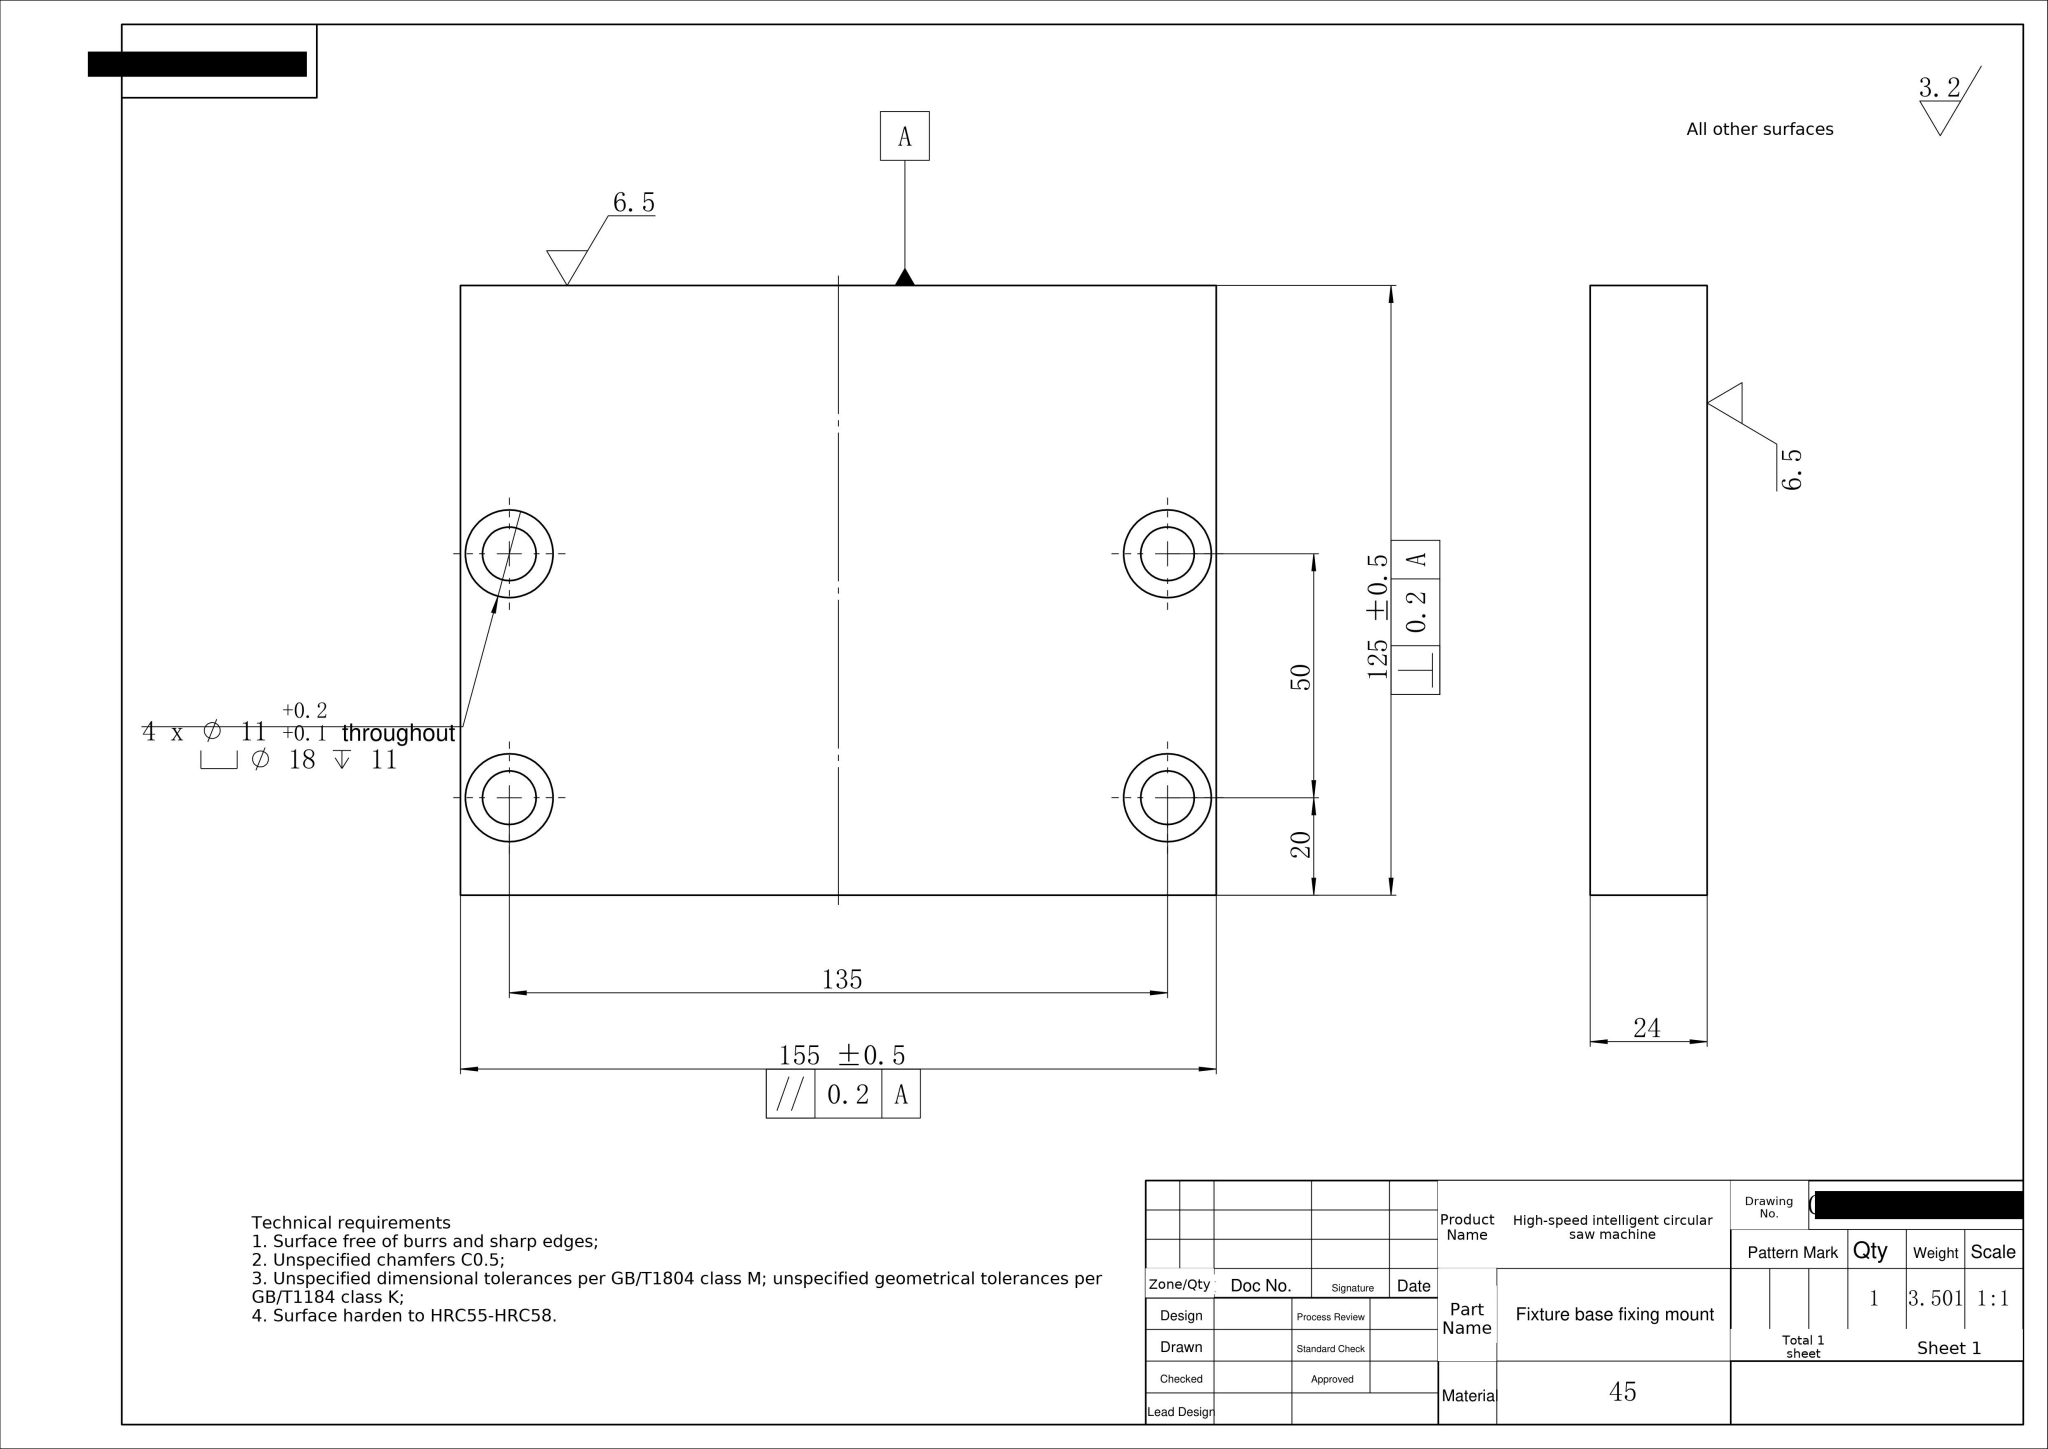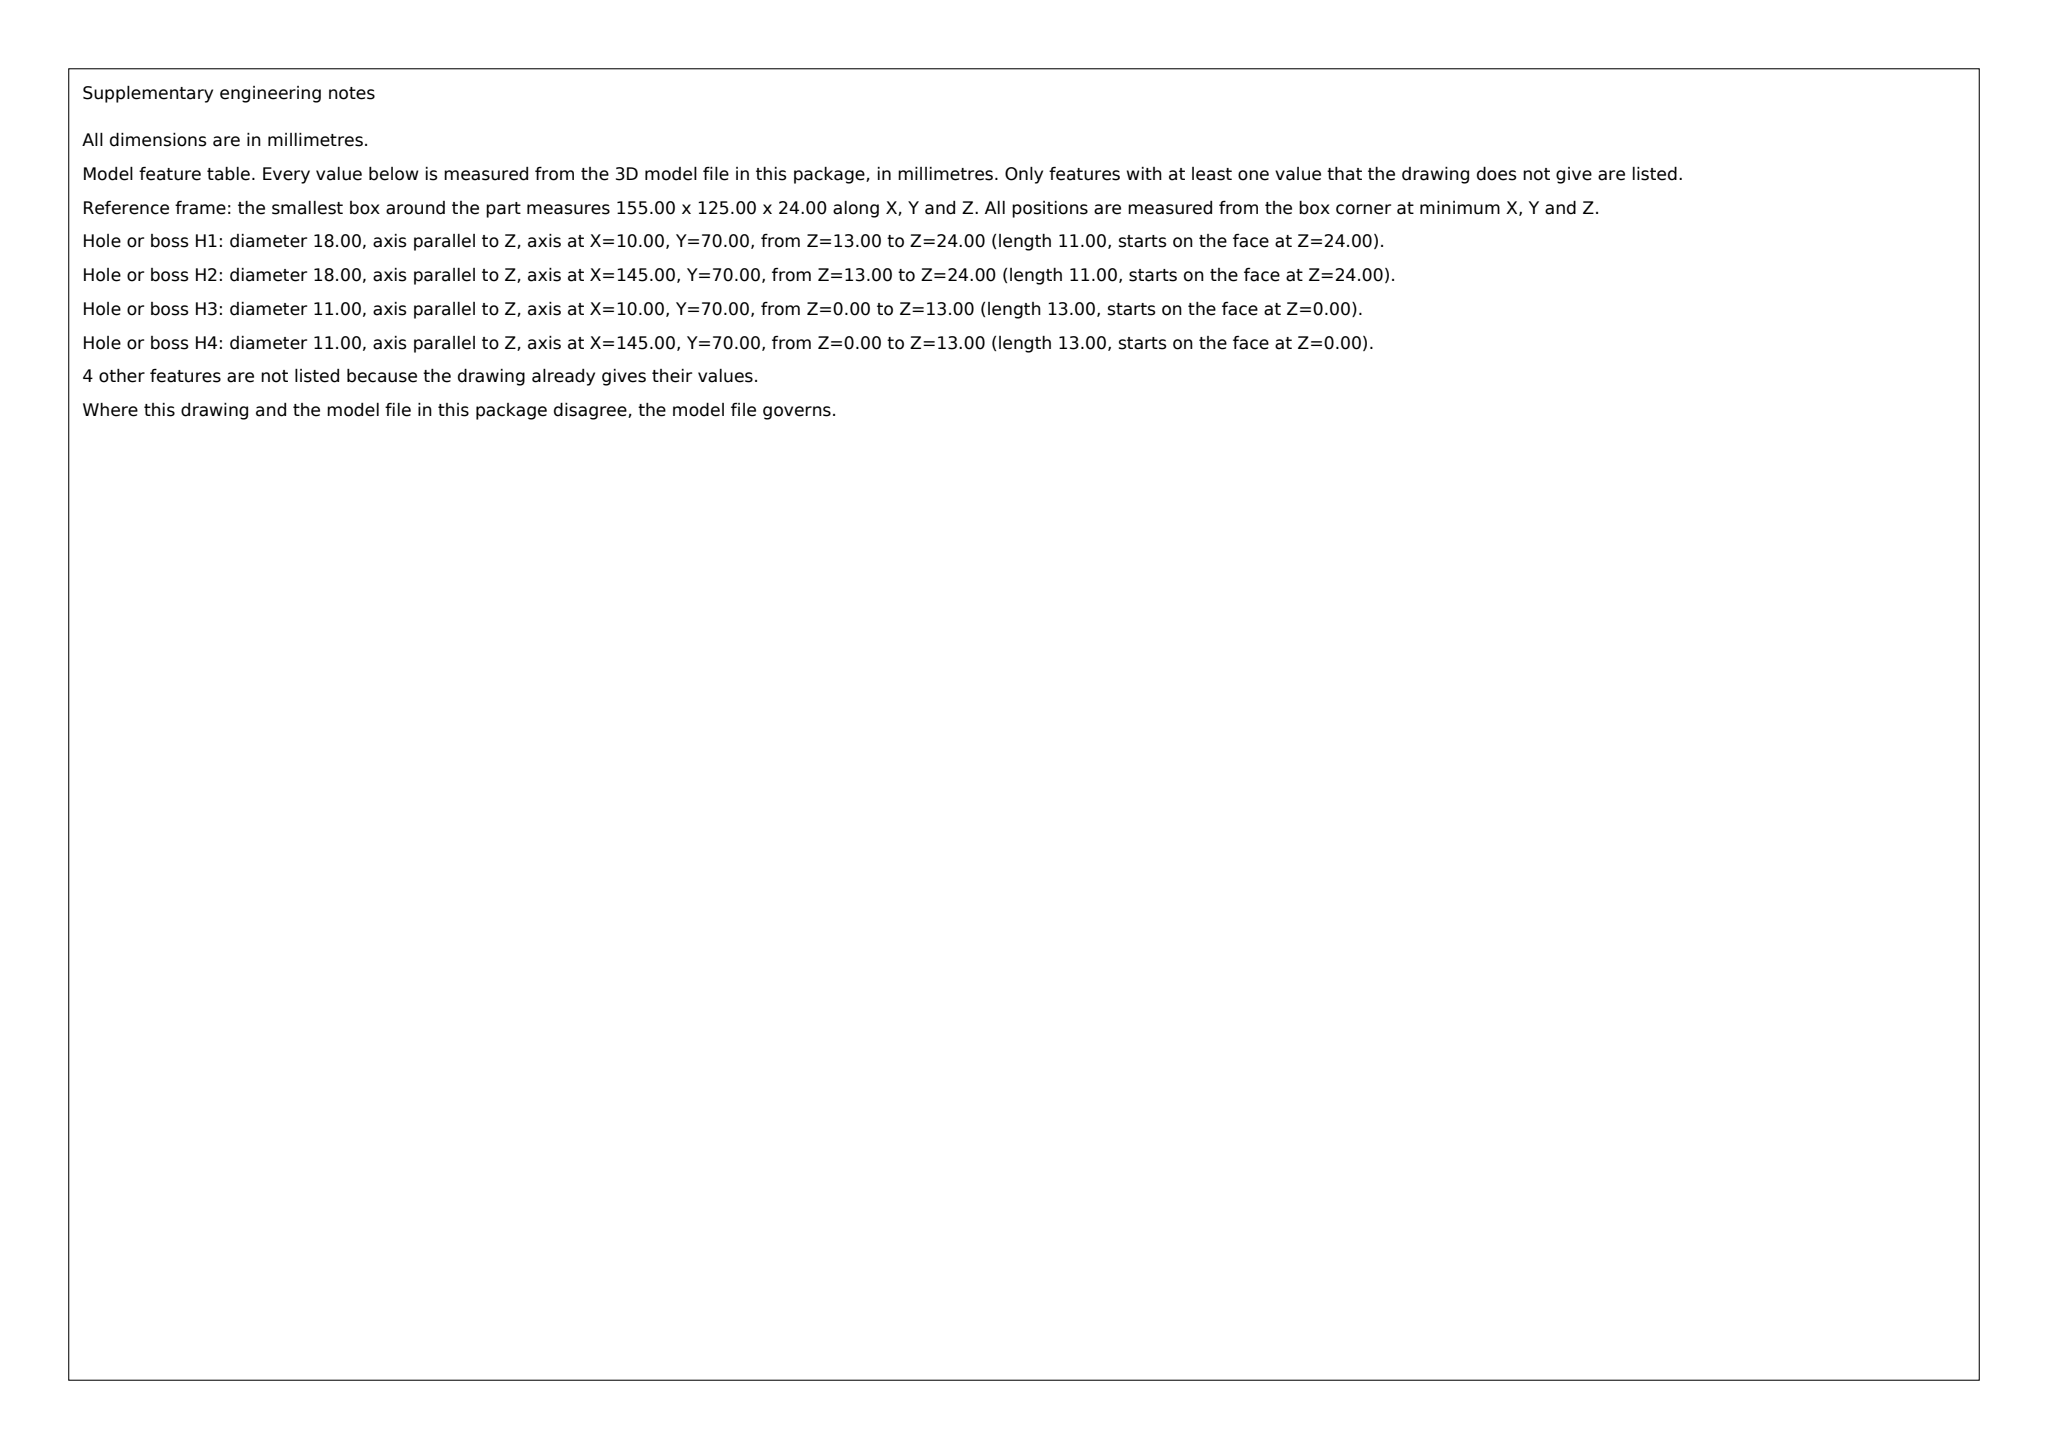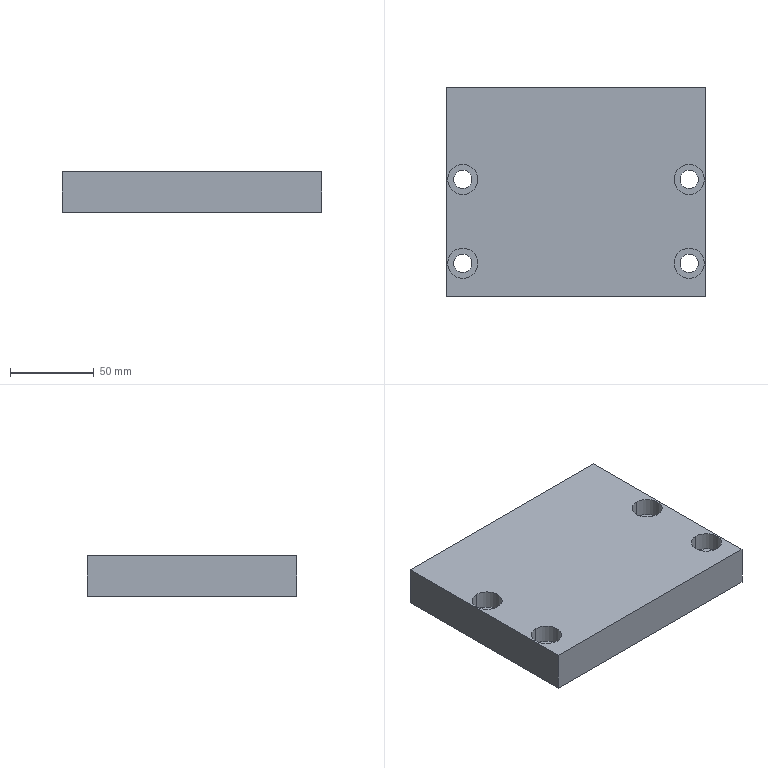Part | SolidWorks | mm | material 45 | 1 solid | 26 faces | box 155 x 125 x 24 mm | volume 448862 mm3 | cylinder 16 | plane 10 | commonest cylinder face diameters 18 x8 11 x8
build123d program:
from build123d import *

# Parameters (mm, degrees)
SKETCH1_W                                          = 24
SKETCH1_H                                          = 125
BOSS_EXTRUDE1_DEPTH                                = 155
HOLE_SIZE_ACCORDING_TO_TYPE_1_OF_HEXAG_D           = 11
HOLE_SIZE_ACCORDING_TO_TYPE_1_OF_HEXAG_CBORE_D     = 18
HOLE_SIZE_ACCORDING_TO_TYPE_1_OF_HEXAG_CBORE_DEPTH = 11


with BuildPart() as part:
    # Sketch1 → Boss-Extrude1 (new body)
    with BuildSketch(Plane(origin=(0, 0, 0), x_dir=(0, 0, -1), z_dir=(1, 0, 0))):
        with Locations((12, 62.5)):
            Rectangle(SKETCH1_W, SKETCH1_H)
    extrude(amount=BOSS_EXTRUDE1_DEPTH)

    # Hole Size _According to_ Type 1 of Hexag (through all)
    with Locations(Plane(origin=(10, 70, 0), x_dir=(1, 0, 0), z_dir=(0, 0, 1))):
        with Locations((0, 0), (0, -50), (135, 0), (135, -50)):
            CounterBoreHole(HOLE_SIZE_ACCORDING_TO_TYPE_1_OF_HEXAG_D / 2, HOLE_SIZE_ACCORDING_TO_TYPE_1_OF_HEXAG_CBORE_D / 2, HOLE_SIZE_ACCORDING_TO_TYPE_1_OF_HEXAG_CBORE_DEPTH)


solid = part.part
STEP:
#1=CARTESIAN_POINT('',(10.,79.,-11.));
#2=VERTEX_POINT('',#1);
#3=CARTESIAN_POINT('',(10.,61.,-11.));
#4=VERTEX_POINT('',#3);
#5=CARTESIAN_POINT('',(10.,70.,-11.));
#6=DIRECTION('',(0.,0.,1.));
#7=DIRECTION('',(0.,-1.,0.));
#8=AXIS2_PLACEMENT_3D('',#5,#6,#7);
#9=CIRCLE('',#8,9.);
#10=EDGE_CURVE('',#2,#4,#9,.T.);
#11=ORIENTED_EDGE('',*,*,#10,.F.);
#12=CARTESIAN_POINT('',(10.,79.,-0.));
#13=VERTEX_POINT('',#12);
#14=CARTESIAN_POINT('',(10.,79.,-0.));
#15=DIRECTION('',(0.,0.,1.));
#16=VECTOR('',#15,1000.);
#17=LINE('',#14,#16);
#18=EDGE_CURVE('',#2,#13,#17,.T.);
#19=ORIENTED_EDGE('',*,*,#18,.T.);
#20=CARTESIAN_POINT('',(10.,61.,0.));
#21=VERTEX_POINT('',#20);
#22=CARTESIAN_POINT('',(10.,70.,0.));
#23=DIRECTION('',(0.,0.,1.));
#24=DIRECTION('',(0.,-1.,0.));
#25=AXIS2_PLACEMENT_3D('',#22,#23,#24);
#26=CIRCLE('',#25,9.);
#27=EDGE_CURVE('',#13,#21,#26,.T.);
#28=ORIENTED_EDGE('',*,*,#27,.T.);
#29=CARTESIAN_POINT('',(10.,61.,0.));
#30=DIRECTION('',(0.,0.,1.));
#31=VECTOR('',#30,1000.);
#32=LINE('',#29,#31);
#33=EDGE_CURVE('',#4,#21,#32,.T.);
#34=ORIENTED_EDGE('',*,*,#33,.F.);
#35=EDGE_LOOP('',(#11,#19,#28,#34));
#36=FACE_OUTER_BOUND('',#35,.T.);
#37=CARTESIAN_POINT('',(10.,70.,0.));
#38=DIRECTION('',(0.,0.,1.));
#39=DIRECTION('',(0.,-1.,0.));
#40=AXIS2_PLACEMENT_3D('',#37,#38,#39);
#41=CYLINDRICAL_SURFACE('',#40,9.);
#42=ADVANCED_FACE('',(#36),#41,.F.);
#43=CARTESIAN_POINT('',(10.,75.5,-24.));
#44=VERTEX_POINT('',#43);
#45=CARTESIAN_POINT('',(10.,64.5,-24.));
#46=VERTEX_POINT('',#45);
#47=CARTESIAN_POINT('',(10.,70.,-24.));
#48=DIRECTION('',(0.,0.,1.));
#49=DIRECTION('',(0.,-1.,0.));
#50=AXIS2_PLACEMENT_3D('',#47,#48,#49);
#51=CIRCLE('',#50,5.5);
#52=EDGE_CURVE('',#44,#46,#51,.T.);
#53=ORIENTED_EDGE('',*,*,#52,.F.);
#54=CARTESIAN_POINT('',(10.,75.5,-11.));
#55=VERTEX_POINT('',#54);
#56=CARTESIAN_POINT('',(10.,75.5,-0.));
#57=DIRECTION('',(0.,0.,1.));
#58=VECTOR('',#57,1000.);
#59=LINE('',#56,#58);
#60=EDGE_CURVE('',#44,#55,#59,.T.);
#61=ORIENTED_EDGE('',*,*,#60,.T.);
#62=CARTESIAN_POINT('',(10.,64.5,-11.));
#63=VERTEX_POINT('',#62);
#64=CARTESIAN_POINT('',(10.,70.,-11.));
#65=DIRECTION('',(0.,0.,1.));
#66=DIRECTION('',(0.,-1.,0.));
#67=AXIS2_PLACEMENT_3D('',#64,#65,#66);
#68=CIRCLE('',#67,5.5);
#69=EDGE_CURVE('',#55,#63,#68,.T.);
#70=ORIENTED_EDGE('',*,*,#69,.T.);
#71=CARTESIAN_POINT('',(10.,64.5,0.));
#72=DIRECTION('',(0.,0.,1.));
#73=VECTOR('',#72,1000.);
#74=LINE('',#71,#73);
#75=EDGE_CURVE('',#46,#63,#74,.T.);
#76=ORIENTED_EDGE('',*,*,#75,.F.);
#77=EDGE_LOOP('',(#53,#61,#70,#76));
#78=FACE_OUTER_BOUND('',#77,.T.);
#79=CARTESIAN_POINT('',(10.,70.,0.));
#80=DIRECTION('',(0.,0.,1.));
#81=DIRECTION('',(0.,-1.,0.));
#82=AXIS2_PLACEMENT_3D('',#79,#80,#81);
#83=CYLINDRICAL_SURFACE('',#82,5.5);
#84=ADVANCED_FACE('',(#78),#83,.F.);
#85=CARTESIAN_POINT('',(10.,29.,-11.));
#86=VERTEX_POINT('',#85);
#87=CARTESIAN_POINT('',(10.,11.,-11.));
#88=VERTEX_POINT('',#87);
#89=CARTESIAN_POINT('',(10.,20.,-11.));
#90=DIRECTION('',(0.,0.,1.));
#91=DIRECTION('',(0.,-1.,0.));
#92=AXIS2_PLACEMENT_3D('',#89,#90,#91);
#93=CIRCLE('',#92,9.);
#94=EDGE_CURVE('',#86,#88,#93,.T.);
#95=ORIENTED_EDGE('',*,*,#94,.F.);
#96=CARTESIAN_POINT('',(10.,29.,-0.));
#97=VERTEX_POINT('',#96);
#98=CARTESIAN_POINT('',(10.,29.,-0.));
#99=DIRECTION('',(0.,0.,1.));
#100=VECTOR('',#99,1000.);
#101=LINE('',#98,#100);
#102=EDGE_CURVE('',#86,#97,#101,.T.);
#103=ORIENTED_EDGE('',*,*,#102,.T.);
#104=CARTESIAN_POINT('',(10.,11.,0.));
#105=VERTEX_POINT('',#104);
#106=CARTESIAN_POINT('',(10.,20.,0.));
#107=DIRECTION('',(0.,0.,1.));
#108=DIRECTION('',(0.,-1.,0.));
#109=AXIS2_PLACEMENT_3D('',#106,#107,#108);
#110=CIRCLE('',#109,9.);
#111=EDGE_CURVE('',#97,#105,#110,.T.);
#112=ORIENTED_EDGE('',*,*,#111,.T.);
#113=CARTESIAN_POINT('',(10.,11.,0.));
#114=DIRECTION('',(0.,0.,1.));
#115=VECTOR('',#114,1000.);
#116=LINE('',#113,#115);
#117=EDGE_CURVE('',#88,#105,#116,.T.);
#118=ORIENTED_EDGE('',*,*,#117,.F.);
#119=EDGE_LOOP('',(#95,#103,#112,#118));
#120=FACE_OUTER_BOUND('',#119,.T.);
#121=CARTESIAN_POINT('',(10.,20.,0.));
#122=DIRECTION('',(0.,0.,1.));
#123=DIRECTION('',(0.,-1.,0.));
#124=AXIS2_PLACEMENT_3D('',#121,#122,#123);
#125=CYLINDRICAL_SURFACE('',#124,9.);
#126=ADVANCED_FACE('',(#120),#125,.F.);
#127=CARTESIAN_POINT('',(10.,25.5,-24.));
#128=VERTEX_POINT('',#127);
#129=CARTESIAN_POINT('',(10.,14.5,-24.));
#130=VERTEX_POINT('',#129);
#131=CARTESIAN_POINT('',(10.,20.,-24.));
#132=DIRECTION('',(0.,0.,1.));
#133=DIRECTION('',(0.,-1.,0.));
#134=AXIS2_PLACEMENT_3D('',#131,#132,#133);
#135=CIRCLE('',#134,5.5);
#136=EDGE_CURVE('',#128,#130,#135,.T.);
#137=ORIENTED_EDGE('',*,*,#136,.F.);
#138=CARTESIAN_POINT('',(10.,25.5,-11.));
#139=VERTEX_POINT('',#138);
#140=CARTESIAN_POINT('',(10.,25.5,-0.));
#141=DIRECTION('',(0.,0.,1.));
#142=VECTOR('',#141,1000.);
#143=LINE('',#140,#142);
#144=EDGE_CURVE('',#128,#139,#143,.T.);
#145=ORIENTED_EDGE('',*,*,#144,.T.);
#146=CARTESIAN_POINT('',(10.,14.5,-11.));
#147=VERTEX_POINT('',#146);
#148=CARTESIAN_POINT('',(10.,20.,-11.));
#149=DIRECTION('',(0.,0.,1.));
#150=DIRECTION('',(0.,-1.,0.));
#151=AXIS2_PLACEMENT_3D('',#148,#149,#150);
#152=CIRCLE('',#151,5.5);
#153=EDGE_CURVE('',#139,#147,#152,.T.);
#154=ORIENTED_EDGE('',*,*,#153,.T.);
#155=CARTESIAN_POINT('',(10.,14.5,0.));
#156=DIRECTION('',(0.,0.,1.));
#157=VECTOR('',#156,1000.);
#158=LINE('',#155,#157);
#159=EDGE_CURVE('',#130,#147,#158,.T.);
#160=ORIENTED_EDGE('',*,*,#159,.F.);
#161=EDGE_LOOP('',(#137,#145,#154,#160));
#162=FACE_OUTER_BOUND('',#161,.T.);
#163=CARTESIAN_POINT('',(10.,20.,0.));
#164=DIRECTION('',(0.,0.,1.));
#165=DIRECTION('',(0.,-1.,0.));
#166=AXIS2_PLACEMENT_3D('',#163,#164,#165);
#167=CYLINDRICAL_SURFACE('',#166,5.5);
#168=ADVANCED_FACE('',(#162),#167,.F.);
#169=CARTESIAN_POINT('',(145.,79.,-11.));
#170=VERTEX_POINT('',#169);
#171=CARTESIAN_POINT('',(145.,61.,-11.));
#172=VERTEX_POINT('',#171);
#173=CARTESIAN_POINT('',(145.,70.,-11.));
#174=DIRECTION('',(0.,0.,1.));
#175=DIRECTION('',(0.,-1.,0.));
#176=AXIS2_PLACEMENT_3D('',#173,#174,#175);
#177=CIRCLE('',#176,9.);
#178=EDGE_CURVE('',#170,#172,#177,.T.);
#179=ORIENTED_EDGE('',*,*,#178,.F.);
#180=CARTESIAN_POINT('',(145.,79.,-0.));
#181=VERTEX_POINT('',#180);
#182=CARTESIAN_POINT('',(145.,79.,-0.));
#183=DIRECTION('',(0.,0.,1.));
#184=VECTOR('',#183,1000.);
#185=LINE('',#182,#184);
#186=EDGE_CURVE('',#170,#181,#185,.T.);
#187=ORIENTED_EDGE('',*,*,#186,.T.);
#188=CARTESIAN_POINT('',(145.,61.,0.));
#189=VERTEX_POINT('',#188);
#190=CARTESIAN_POINT('',(145.,70.,0.));
#191=DIRECTION('',(0.,0.,1.));
#192=DIRECTION('',(0.,-1.,0.));
#193=AXIS2_PLACEMENT_3D('',#190,#191,#192);
#194=CIRCLE('',#193,9.);
#195=EDGE_CURVE('',#181,#189,#194,.T.);
#196=ORIENTED_EDGE('',*,*,#195,.T.);
#197=CARTESIAN_POINT('',(145.,61.,0.));
#198=DIRECTION('',(0.,0.,1.));
#199=VECTOR('',#198,1000.);
#200=LINE('',#197,#199);
#201=EDGE_CURVE('',#172,#189,#200,.T.);
#202=ORIENTED_EDGE('',*,*,#201,.F.);
#203=EDGE_LOOP('',(#179,#187,#196,#202));
#204=FACE_OUTER_BOUND('',#203,.T.);
#205=CARTESIAN_POINT('',(145.,70.,0.));
#206=DIRECTION('',(0.,0.,1.));
#207=DIRECTION('',(0.,-1.,0.));
#208=AXIS2_PLACEMENT_3D('',#205,#206,#207);
#209=CYLINDRICAL_SURFACE('',#208,9.);
#210=ADVANCED_FACE('',(#204),#209,.F.);
#211=CARTESIAN_POINT('',(145.,75.5,-24.));
#212=VERTEX_POINT('',#211);
#213=CARTESIAN_POINT('',(145.,64.5,-24.));
#214=VERTEX_POINT('',#213);
#215=CARTESIAN_POINT('',(145.,70.,-24.));
#216=DIRECTION('',(0.,0.,1.));
#217=DIRECTION('',(0.,-1.,0.));
#218=AXIS2_PLACEMENT_3D('',#215,#216,#217);
#219=CIRCLE('',#218,5.5);
#220=EDGE_CURVE('',#212,#214,#219,.T.);
#221=ORIENTED_EDGE('',*,*,#220,.F.);
#222=CARTESIAN_POINT('',(145.,75.5,-11.));
#223=VERTEX_POINT('',#222);
#224=CARTESIAN_POINT('',(145.,75.5,-0.));
#225=DIRECTION('',(0.,0.,1.));
#226=VECTOR('',#225,1000.);
#227=LINE('',#224,#226);
#228=EDGE_CURVE('',#212,#223,#227,.T.);
#229=ORIENTED_EDGE('',*,*,#228,.T.);
#230=CARTESIAN_POINT('',(145.,64.5,-11.));
#231=VERTEX_POINT('',#230);
#232=CARTESIAN_POINT('',(145.,70.,-11.));
#233=DIRECTION('',(0.,0.,1.));
#234=DIRECTION('',(0.,-1.,0.));
#235=AXIS2_PLACEMENT_3D('',#232,#233,#234);
#236=CIRCLE('',#235,5.5);
#237=EDGE_CURVE('',#223,#231,#236,.T.);
#238=ORIENTED_EDGE('',*,*,#237,.T.);
#239=CARTESIAN_POINT('',(145.,64.5,0.));
#240=DIRECTION('',(0.,0.,1.));
#241=VECTOR('',#240,1000.);
#242=LINE('',#239,#241);
#243=EDGE_CURVE('',#214,#231,#242,.T.);
#244=ORIENTED_EDGE('',*,*,#243,.F.);
#245=EDGE_LOOP('',(#221,#229,#238,#244));
#246=FACE_OUTER_BOUND('',#245,.T.);
#247=CARTESIAN_POINT('',(145.,70.,0.));
#248=DIRECTION('',(0.,0.,1.));
#249=DIRECTION('',(0.,-1.,0.));
#250=AXIS2_PLACEMENT_3D('',#247,#248,#249);
#251=CYLINDRICAL_SURFACE('',#250,5.5);
#252=ADVANCED_FACE('',(#246),#251,.F.);
#253=CARTESIAN_POINT('',(145.,29.,-11.));
#254=VERTEX_POINT('',#253);
#255=CARTESIAN_POINT('',(145.,11.,-11.));
#256=VERTEX_POINT('',#255);
#257=CARTESIAN_POINT('',(145.,20.,-11.));
#258=DIRECTION('',(0.,0.,1.));
#259=DIRECTION('',(0.,-1.,0.));
#260=AXIS2_PLACEMENT_3D('',#257,#258,#259);
#261=CIRCLE('',#260,9.);
#262=EDGE_CURVE('',#254,#256,#261,.T.);
#263=ORIENTED_EDGE('',*,*,#262,.F.);
#264=CARTESIAN_POINT('',(145.,29.,-0.));
#265=VERTEX_POINT('',#264);
#266=CARTESIAN_POINT('',(145.,29.,-0.));
#267=DIRECTION('',(0.,0.,1.));
#268=VECTOR('',#267,1000.);
#269=LINE('',#266,#268);
#270=EDGE_CURVE('',#254,#265,#269,.T.);
#271=ORIENTED_EDGE('',*,*,#270,.T.);
#272=CARTESIAN_POINT('',(145.,11.,0.));
#273=VERTEX_POINT('',#272);
#274=CARTESIAN_POINT('',(145.,20.,0.));
#275=DIRECTION('',(0.,0.,1.));
#276=DIRECTION('',(0.,-1.,0.));
#277=AXIS2_PLACEMENT_3D('',#274,#275,#276);
#278=CIRCLE('',#277,9.);
#279=EDGE_CURVE('',#265,#273,#278,.T.);
#280=ORIENTED_EDGE('',*,*,#279,.T.);
#281=CARTESIAN_POINT('',(145.,11.,0.));
#282=DIRECTION('',(0.,0.,1.));
#283=VECTOR('',#282,1000.);
#284=LINE('',#281,#283);
#285=EDGE_CURVE('',#256,#273,#284,.T.);
#286=ORIENTED_EDGE('',*,*,#285,.F.);
#287=EDGE_LOOP('',(#263,#271,#280,#286));
#288=FACE_OUTER_BOUND('',#287,.T.);
#289=CARTESIAN_POINT('',(145.,20.,0.));
#290=DIRECTION('',(0.,0.,1.));
#291=DIRECTION('',(0.,-1.,0.));
#292=AXIS2_PLACEMENT_3D('',#289,#290,#291);
#293=CYLINDRICAL_SURFACE('',#292,9.);
#294=ADVANCED_FACE('',(#288),#293,.F.);
#295=CARTESIAN_POINT('',(145.,25.5,-24.));
#296=VERTEX_POINT('',#295);
#297=CARTESIAN_POINT('',(145.,14.5,-24.));
#298=VERTEX_POINT('',#297);
#299=CARTESIAN_POINT('',(145.,20.,-24.));
#300=DIRECTION('',(0.,0.,1.));
#301=DIRECTION('',(0.,-1.,0.));
#302=AXIS2_PLACEMENT_3D('',#299,#300,#301);
#303=CIRCLE('',#302,5.5);
#304=EDGE_CURVE('',#296,#298,#303,.T.);
#305=ORIENTED_EDGE('',*,*,#304,.F.);
#306=CARTESIAN_POINT('',(145.,25.5,-11.));
#307=VERTEX_POINT('',#306);
#308=CARTESIAN_POINT('',(145.,25.5,-0.));
#309=DIRECTION('',(0.,0.,1.));
#310=VECTOR('',#309,1000.);
#311=LINE('',#308,#310);
#312=EDGE_CURVE('',#296,#307,#311,.T.);
#313=ORIENTED_EDGE('',*,*,#312,.T.);
#314=CARTESIAN_POINT('',(145.,14.5,-11.));
#315=VERTEX_POINT('',#314);
#316=CARTESIAN_POINT('',(145.,20.,-11.));
#317=DIRECTION('',(0.,0.,1.));
#318=DIRECTION('',(0.,-1.,0.));
#319=AXIS2_PLACEMENT_3D('',#316,#317,#318);
#320=CIRCLE('',#319,5.5);
#321=EDGE_CURVE('',#307,#315,#320,.T.);
#322=ORIENTED_EDGE('',*,*,#321,.T.);
#323=CARTESIAN_POINT('',(145.,14.5,0.));
#324=DIRECTION('',(0.,0.,1.));
#325=VECTOR('',#324,1000.);
#326=LINE('',#323,#325);
#327=EDGE_CURVE('',#298,#315,#326,.T.);
#328=ORIENTED_EDGE('',*,*,#327,.F.);
#329=EDGE_LOOP('',(#305,#313,#322,#328));
#330=FACE_OUTER_BOUND('',#329,.T.);
#331=CARTESIAN_POINT('',(145.,20.,0.));
#332=DIRECTION('',(0.,0.,1.));
#333=DIRECTION('',(0.,-1.,0.));
#334=AXIS2_PLACEMENT_3D('',#331,#332,#333);
#335=CYLINDRICAL_SURFACE('',#334,5.5);
#336=ADVANCED_FACE('',(#330),#335,.F.);
#337=CARTESIAN_POINT('',(10.,70.,0.));
#338=DIRECTION('',(0.,0.,1.));
#339=DIRECTION('',(0.,-1.,0.));
#340=AXIS2_PLACEMENT_3D('',#337,#338,#339);
#341=CIRCLE('',#340,9.);
#342=EDGE_CURVE('',#21,#13,#341,.T.);
#343=ORIENTED_EDGE('',*,*,#342,.F.);
#344=ORIENTED_EDGE('',*,*,#27,.F.);
#345=EDGE_LOOP('',(#343,#344));
#346=FACE_BOUND('',#345,.T.);
#347=CARTESIAN_POINT('',(10.,20.,0.));
#348=DIRECTION('',(0.,0.,1.));
#349=DIRECTION('',(0.,-1.,0.));
#350=AXIS2_PLACEMENT_3D('',#347,#348,#349);
#351=CIRCLE('',#350,9.);
#352=EDGE_CURVE('',#105,#97,#351,.T.);
#353=ORIENTED_EDGE('',*,*,#352,.F.);
#354=ORIENTED_EDGE('',*,*,#111,.F.);
#355=EDGE_LOOP('',(#353,#354));
#356=FACE_BOUND('',#355,.T.);
#357=CARTESIAN_POINT('',(145.,70.,0.));
#358=DIRECTION('',(0.,0.,1.));
#359=DIRECTION('',(0.,-1.,0.));
#360=AXIS2_PLACEMENT_3D('',#357,#358,#359);
#361=CIRCLE('',#360,9.);
#362=EDGE_CURVE('',#189,#181,#361,.T.);
#363=ORIENTED_EDGE('',*,*,#362,.F.);
#364=ORIENTED_EDGE('',*,*,#195,.F.);
#365=EDGE_LOOP('',(#363,#364));
#366=FACE_BOUND('',#365,.T.);
#367=CARTESIAN_POINT('',(145.,20.,0.));
#368=DIRECTION('',(0.,0.,1.));
#369=DIRECTION('',(0.,-1.,0.));
#370=AXIS2_PLACEMENT_3D('',#367,#368,#369);
#371=CIRCLE('',#370,9.);
#372=EDGE_CURVE('',#273,#265,#371,.T.);
#373=ORIENTED_EDGE('',*,*,#372,.F.);
#374=ORIENTED_EDGE('',*,*,#279,.F.);
#375=EDGE_LOOP('',(#373,#374));
#376=FACE_BOUND('',#375,.T.);
#377=CARTESIAN_POINT('',(0.,125.,-0.));
#378=VERTEX_POINT('',#377);
#379=CARTESIAN_POINT('',(0.,0.,0.));
#380=VERTEX_POINT('',#379);
#381=CARTESIAN_POINT('',(0.,125.,-0.));
#382=DIRECTION('',(0.,-1.,0.));
#383=VECTOR('',#382,1000.);
#384=LINE('',#381,#383);
#385=EDGE_CURVE('',#378,#380,#384,.T.);
#386=ORIENTED_EDGE('',*,*,#385,.T.);
#387=CARTESIAN_POINT('',(155.,0.,0.));
#388=VERTEX_POINT('',#387);
#389=CARTESIAN_POINT('',(155.,0.,0.));
#390=DIRECTION('',(-1.,0.,0.));
#391=VECTOR('',#390,1000.);
#392=LINE('',#389,#391);
#393=EDGE_CURVE('',#388,#380,#392,.T.);
#394=ORIENTED_EDGE('',*,*,#393,.F.);
#395=CARTESIAN_POINT('',(155.,125.,-0.));
#396=VERTEX_POINT('',#395);
#397=CARTESIAN_POINT('',(155.,125.,-0.));
#398=DIRECTION('',(0.,-1.,0.));
#399=VECTOR('',#398,1000.);
#400=LINE('',#397,#399);
#401=EDGE_CURVE('',#396,#388,#400,.T.);
#402=ORIENTED_EDGE('',*,*,#401,.F.);
#403=CARTESIAN_POINT('',(155.,125.,-0.));
#404=DIRECTION('',(-1.,0.,0.));
#405=VECTOR('',#404,1000.);
#406=LINE('',#403,#405);
#407=EDGE_CURVE('',#396,#378,#406,.T.);
#408=ORIENTED_EDGE('',*,*,#407,.T.);
#409=EDGE_LOOP('',(#386,#394,#402,#408));
#410=FACE_OUTER_BOUND('',#409,.T.);
#411=CARTESIAN_POINT('',(155.,125.,-0.));
#412=DIRECTION('',(0.,-0.,-1.));
#413=DIRECTION('',(0.,1.,-0.));
#414=AXIS2_PLACEMENT_3D('',#411,#412,#413);
#415=PLANE('',#414);
#416=ADVANCED_FACE('',(#346,#356,#366,#376,#410),#415,.F.);
#417=CARTESIAN_POINT('',(0.,0.,-24.));
#418=VERTEX_POINT('',#417);
#419=CARTESIAN_POINT('',(0.,0.,0.));
#420=DIRECTION('',(0.,0.,-1.));
#421=VECTOR('',#420,1000.);
#422=LINE('',#419,#421);
#423=EDGE_CURVE('',#380,#418,#422,.T.);
#424=ORIENTED_EDGE('',*,*,#423,.T.);
#425=CARTESIAN_POINT('',(155.,0.,-24.));
#426=VERTEX_POINT('',#425);
#427=CARTESIAN_POINT('',(155.,0.,-24.));
#428=DIRECTION('',(-1.,0.,0.));
#429=VECTOR('',#428,1000.);
#430=LINE('',#427,#429);
#431=EDGE_CURVE('',#426,#418,#430,.T.);
#432=ORIENTED_EDGE('',*,*,#431,.F.);
#433=CARTESIAN_POINT('',(155.,0.,0.));
#434=DIRECTION('',(0.,0.,-1.));
#435=VECTOR('',#434,1000.);
#436=LINE('',#433,#435);
#437=EDGE_CURVE('',#388,#426,#436,.T.);
#438=ORIENTED_EDGE('',*,*,#437,.F.);
#439=ORIENTED_EDGE('',*,*,#393,.T.);
#440=EDGE_LOOP('',(#424,#432,#438,#439));
#441=FACE_OUTER_BOUND('',#440,.T.);
#442=CARTESIAN_POINT('',(155.,0.,0.));
#443=DIRECTION('',(0.,1.,0.));
#444=DIRECTION('',(0.,0.,1.));
#445=AXIS2_PLACEMENT_3D('',#442,#443,#444);
#446=PLANE('',#445);
#447=ADVANCED_FACE('',(#441),#446,.F.);
#448=CARTESIAN_POINT('',(10.,70.,-24.));
#449=DIRECTION('',(0.,0.,1.));
#450=DIRECTION('',(0.,-1.,0.));
#451=AXIS2_PLACEMENT_3D('',#448,#449,#450);
#452=CIRCLE('',#451,5.5);
#453=EDGE_CURVE('',#46,#44,#452,.T.);
#454=ORIENTED_EDGE('',*,*,#453,.T.);
#455=ORIENTED_EDGE('',*,*,#52,.T.);
#456=EDGE_LOOP('',(#454,#455));
#457=FACE_BOUND('',#456,.T.);
#458=CARTESIAN_POINT('',(10.,20.,-24.));
#459=DIRECTION('',(0.,0.,1.));
#460=DIRECTION('',(0.,-1.,0.));
#461=AXIS2_PLACEMENT_3D('',#458,#459,#460);
#462=CIRCLE('',#461,5.5);
#463=EDGE_CURVE('',#130,#128,#462,.T.);
#464=ORIENTED_EDGE('',*,*,#463,.T.);
#465=ORIENTED_EDGE('',*,*,#136,.T.);
#466=EDGE_LOOP('',(#464,#465));
#467=FACE_BOUND('',#466,.T.);
#468=CARTESIAN_POINT('',(145.,70.,-24.));
#469=DIRECTION('',(0.,0.,1.));
#470=DIRECTION('',(0.,-1.,0.));
#471=AXIS2_PLACEMENT_3D('',#468,#469,#470);
#472=CIRCLE('',#471,5.5);
#473=EDGE_CURVE('',#214,#212,#472,.T.);
#474=ORIENTED_EDGE('',*,*,#473,.T.);
#475=ORIENTED_EDGE('',*,*,#220,.T.);
#476=EDGE_LOOP('',(#474,#475));
#477=FACE_BOUND('',#476,.T.);
#478=CARTESIAN_POINT('',(145.,20.,-24.));
#479=DIRECTION('',(0.,0.,1.));
#480=DIRECTION('',(0.,-1.,0.));
#481=AXIS2_PLACEMENT_3D('',#478,#479,#480);
#482=CIRCLE('',#481,5.5);
#483=EDGE_CURVE('',#298,#296,#482,.T.);
#484=ORIENTED_EDGE('',*,*,#483,.T.);
#485=ORIENTED_EDGE('',*,*,#304,.T.);
#486=EDGE_LOOP('',(#484,#485));
#487=FACE_BOUND('',#486,.T.);
#488=CARTESIAN_POINT('',(0.,125.,-24.));
#489=VERTEX_POINT('',#488);
#490=CARTESIAN_POINT('',(0.,0.,-24.));
#491=DIRECTION('',(0.,1.,0.));
#492=VECTOR('',#491,1000.);
#493=LINE('',#490,#492);
#494=EDGE_CURVE('',#418,#489,#493,.T.);
#495=ORIENTED_EDGE('',*,*,#494,.T.);
#496=CARTESIAN_POINT('',(155.,125.,-24.));
#497=VERTEX_POINT('',#496);
#498=CARTESIAN_POINT('',(155.,125.,-24.));
#499=DIRECTION('',(-1.,0.,0.));
#500=VECTOR('',#499,1000.);
#501=LINE('',#498,#500);
#502=EDGE_CURVE('',#497,#489,#501,.T.);
#503=ORIENTED_EDGE('',*,*,#502,.F.);
#504=CARTESIAN_POINT('',(155.,0.,-24.));
#505=DIRECTION('',(0.,1.,0.));
#506=VECTOR('',#505,1000.);
#507=LINE('',#504,#506);
#508=EDGE_CURVE('',#426,#497,#507,.T.);
#509=ORIENTED_EDGE('',*,*,#508,.F.);
#510=ORIENTED_EDGE('',*,*,#431,.T.);
#511=EDGE_LOOP('',(#495,#503,#509,#510));
#512=FACE_OUTER_BOUND('',#511,.T.);
#513=CARTESIAN_POINT('',(155.,0.,-24.));
#514=DIRECTION('',(0.,0.,1.));
#515=DIRECTION('',(1.,0.,0.));
#516=AXIS2_PLACEMENT_3D('',#513,#514,#515);
#517=PLANE('',#516);
#518=ADVANCED_FACE('',(#457,#467,#477,#487,#512),#517,.F.);
#519=CARTESIAN_POINT('',(0.,125.,-0.));
#520=DIRECTION('',(0.,0.,1.));
#521=VECTOR('',#520,1000.);
#522=LINE('',#519,#521);
#523=EDGE_CURVE('',#489,#378,#522,.T.);
#524=ORIENTED_EDGE('',*,*,#523,.T.);
#525=ORIENTED_EDGE('',*,*,#407,.F.);
#526=CARTESIAN_POINT('',(155.,125.,-0.));
#527=DIRECTION('',(0.,0.,1.));
#528=VECTOR('',#527,1000.);
#529=LINE('',#526,#528);
#530=EDGE_CURVE('',#497,#396,#529,.T.);
#531=ORIENTED_EDGE('',*,*,#530,.F.);
#532=ORIENTED_EDGE('',*,*,#502,.T.);
#533=EDGE_LOOP('',(#524,#525,#531,#532));
#534=FACE_OUTER_BOUND('',#533,.T.);
#535=CARTESIAN_POINT('',(155.,125.,-0.));
#536=DIRECTION('',(0.,-1.,0.));
#537=DIRECTION('',(0.,0.,-1.));
#538=AXIS2_PLACEMENT_3D('',#535,#536,#537);
#539=PLANE('',#538);
#540=ADVANCED_FACE('',(#534),#539,.F.);
#541=ORIENTED_EDGE('',*,*,#401,.T.);
#542=ORIENTED_EDGE('',*,*,#437,.T.);
#543=ORIENTED_EDGE('',*,*,#508,.T.);
#544=ORIENTED_EDGE('',*,*,#530,.T.);
#545=EDGE_LOOP('',(#541,#542,#543,#544));
#546=FACE_OUTER_BOUND('',#545,.T.);
#547=CARTESIAN_POINT('',(155.,0.,0.));
#548=DIRECTION('',(1.,0.,0.));
#549=DIRECTION('',(0.,0.,-1.));
#550=AXIS2_PLACEMENT_3D('',#547,#548,#549);
#551=PLANE('',#550);
#552=ADVANCED_FACE('',(#546),#551,.T.);
#553=ORIENTED_EDGE('',*,*,#385,.F.);
#554=ORIENTED_EDGE('',*,*,#523,.F.);
#555=ORIENTED_EDGE('',*,*,#494,.F.);
#556=ORIENTED_EDGE('',*,*,#423,.F.);
#557=EDGE_LOOP('',(#553,#554,#555,#556));
#558=FACE_OUTER_BOUND('',#557,.T.);
#559=CARTESIAN_POINT('',(0.,0.,0.));
#560=DIRECTION('',(1.,0.,0.));
#561=DIRECTION('',(0.,0.,-1.));
#562=AXIS2_PLACEMENT_3D('',#559,#560,#561);
#563=PLANE('',#562);
#564=ADVANCED_FACE('',(#558),#563,.F.);
#565=ORIENTED_EDGE('',*,*,#312,.F.);
#566=ORIENTED_EDGE('',*,*,#483,.F.);
#567=ORIENTED_EDGE('',*,*,#327,.T.);
#568=CARTESIAN_POINT('',(145.,20.,-11.));
#569=DIRECTION('',(0.,0.,1.));
#570=DIRECTION('',(0.,-1.,0.));
#571=AXIS2_PLACEMENT_3D('',#568,#569,#570);
#572=CIRCLE('',#571,5.5);
#573=EDGE_CURVE('',#315,#307,#572,.T.);
#574=ORIENTED_EDGE('',*,*,#573,.T.);
#575=EDGE_LOOP('',(#565,#566,#567,#574));
#576=FACE_OUTER_BOUND('',#575,.T.);
#577=CARTESIAN_POINT('',(145.,20.,0.));
#578=DIRECTION('',(0.,0.,1.));
#579=DIRECTION('',(0.,-1.,0.));
#580=AXIS2_PLACEMENT_3D('',#577,#578,#579);
#581=CYLINDRICAL_SURFACE('',#580,5.5);
#582=ADVANCED_FACE('',(#576),#581,.F.);
#583=ORIENTED_EDGE('',*,*,#573,.F.);
#584=ORIENTED_EDGE('',*,*,#321,.F.);
#585=EDGE_LOOP('',(#583,#584));
#586=FACE_BOUND('',#585,.T.);
#587=CARTESIAN_POINT('',(145.,20.,-11.));
#588=DIRECTION('',(0.,0.,1.));
#589=DIRECTION('',(0.,-1.,0.));
#590=AXIS2_PLACEMENT_3D('',#587,#588,#589);
#591=CIRCLE('',#590,9.);
#592=EDGE_CURVE('',#256,#254,#591,.T.);
#593=ORIENTED_EDGE('',*,*,#592,.T.);
#594=ORIENTED_EDGE('',*,*,#262,.T.);
#595=EDGE_LOOP('',(#593,#594));
#596=FACE_OUTER_BOUND('',#595,.T.);
#597=CARTESIAN_POINT('',(150.5,20.,-11.));
#598=DIRECTION('',(0.,-0.,-1.));
#599=DIRECTION('',(0.,1.,-0.));
#600=AXIS2_PLACEMENT_3D('',#597,#598,#599);
#601=PLANE('',#600);
#602=ADVANCED_FACE('',(#586,#596),#601,.F.);
#603=ORIENTED_EDGE('',*,*,#270,.F.);
#604=ORIENTED_EDGE('',*,*,#592,.F.);
#605=ORIENTED_EDGE('',*,*,#285,.T.);
#606=ORIENTED_EDGE('',*,*,#372,.T.);
#607=EDGE_LOOP('',(#603,#604,#605,#606));
#608=FACE_OUTER_BOUND('',#607,.T.);
#609=CARTESIAN_POINT('',(145.,20.,0.));
#610=DIRECTION('',(0.,0.,1.));
#611=DIRECTION('',(0.,-1.,0.));
#612=AXIS2_PLACEMENT_3D('',#609,#610,#611);
#613=CYLINDRICAL_SURFACE('',#612,9.);
#614=ADVANCED_FACE('',(#608),#613,.F.);
#615=ORIENTED_EDGE('',*,*,#228,.F.);
#616=ORIENTED_EDGE('',*,*,#473,.F.);
#617=ORIENTED_EDGE('',*,*,#243,.T.);
#618=CARTESIAN_POINT('',(145.,70.,-11.));
#619=DIRECTION('',(0.,0.,1.));
#620=DIRECTION('',(0.,-1.,0.));
#621=AXIS2_PLACEMENT_3D('',#618,#619,#620);
#622=CIRCLE('',#621,5.5);
#623=EDGE_CURVE('',#231,#223,#622,.T.);
#624=ORIENTED_EDGE('',*,*,#623,.T.);
#625=EDGE_LOOP('',(#615,#616,#617,#624));
#626=FACE_OUTER_BOUND('',#625,.T.);
#627=CARTESIAN_POINT('',(145.,70.,0.));
#628=DIRECTION('',(0.,0.,1.));
#629=DIRECTION('',(0.,-1.,0.));
#630=AXIS2_PLACEMENT_3D('',#627,#628,#629);
#631=CYLINDRICAL_SURFACE('',#630,5.5);
#632=ADVANCED_FACE('',(#626),#631,.F.);
#633=ORIENTED_EDGE('',*,*,#623,.F.);
#634=ORIENTED_EDGE('',*,*,#237,.F.);
#635=EDGE_LOOP('',(#633,#634));
#636=FACE_BOUND('',#635,.T.);
#637=CARTESIAN_POINT('',(145.,70.,-11.));
#638=DIRECTION('',(0.,0.,1.));
#639=DIRECTION('',(0.,-1.,0.));
#640=AXIS2_PLACEMENT_3D('',#637,#638,#639);
#641=CIRCLE('',#640,9.);
#642=EDGE_CURVE('',#172,#170,#641,.T.);
#643=ORIENTED_EDGE('',*,*,#642,.T.);
#644=ORIENTED_EDGE('',*,*,#178,.T.);
#645=EDGE_LOOP('',(#643,#644));
#646=FACE_OUTER_BOUND('',#645,.T.);
#647=CARTESIAN_POINT('',(150.5,70.,-11.));
#648=DIRECTION('',(0.,-0.,-1.));
#649=DIRECTION('',(0.,1.,-0.));
#650=AXIS2_PLACEMENT_3D('',#647,#648,#649);
#651=PLANE('',#650);
#652=ADVANCED_FACE('',(#636,#646),#651,.F.);
#653=ORIENTED_EDGE('',*,*,#186,.F.);
#654=ORIENTED_EDGE('',*,*,#642,.F.);
#655=ORIENTED_EDGE('',*,*,#201,.T.);
#656=ORIENTED_EDGE('',*,*,#362,.T.);
#657=EDGE_LOOP('',(#653,#654,#655,#656));
#658=FACE_OUTER_BOUND('',#657,.T.);
#659=CARTESIAN_POINT('',(145.,70.,0.));
#660=DIRECTION('',(0.,0.,1.));
#661=DIRECTION('',(0.,-1.,0.));
#662=AXIS2_PLACEMENT_3D('',#659,#660,#661);
#663=CYLINDRICAL_SURFACE('',#662,9.);
#664=ADVANCED_FACE('',(#658),#663,.F.);
#665=ORIENTED_EDGE('',*,*,#144,.F.);
#666=ORIENTED_EDGE('',*,*,#463,.F.);
#667=ORIENTED_EDGE('',*,*,#159,.T.);
#668=CARTESIAN_POINT('',(10.,20.,-11.));
#669=DIRECTION('',(0.,0.,1.));
#670=DIRECTION('',(0.,-1.,0.));
#671=AXIS2_PLACEMENT_3D('',#668,#669,#670);
#672=CIRCLE('',#671,5.5);
#673=EDGE_CURVE('',#147,#139,#672,.T.);
#674=ORIENTED_EDGE('',*,*,#673,.T.);
#675=EDGE_LOOP('',(#665,#666,#667,#674));
#676=FACE_OUTER_BOUND('',#675,.T.);
#677=CARTESIAN_POINT('',(10.,20.,0.));
#678=DIRECTION('',(0.,0.,1.));
#679=DIRECTION('',(0.,-1.,0.));
#680=AXIS2_PLACEMENT_3D('',#677,#678,#679);
#681=CYLINDRICAL_SURFACE('',#680,5.5);
#682=ADVANCED_FACE('',(#676),#681,.F.);
#683=ORIENTED_EDGE('',*,*,#673,.F.);
#684=ORIENTED_EDGE('',*,*,#153,.F.);
#685=EDGE_LOOP('',(#683,#684));
#686=FACE_BOUND('',#685,.T.);
#687=CARTESIAN_POINT('',(10.,20.,-11.));
#688=DIRECTION('',(0.,0.,1.));
#689=DIRECTION('',(0.,-1.,0.));
#690=AXIS2_PLACEMENT_3D('',#687,#688,#689);
#691=CIRCLE('',#690,9.);
#692=EDGE_CURVE('',#88,#86,#691,.T.);
#693=ORIENTED_EDGE('',*,*,#692,.T.);
#694=ORIENTED_EDGE('',*,*,#94,.T.);
#695=EDGE_LOOP('',(#693,#694));
#696=FACE_OUTER_BOUND('',#695,.T.);
#697=CARTESIAN_POINT('',(15.5,20.,-11.));
#698=DIRECTION('',(0.,-0.,-1.));
#699=DIRECTION('',(0.,1.,-0.));
#700=AXIS2_PLACEMENT_3D('',#697,#698,#699);
#701=PLANE('',#700);
#702=ADVANCED_FACE('',(#686,#696),#701,.F.);
#703=ORIENTED_EDGE('',*,*,#102,.F.);
#704=ORIENTED_EDGE('',*,*,#692,.F.);
#705=ORIENTED_EDGE('',*,*,#117,.T.);
#706=ORIENTED_EDGE('',*,*,#352,.T.);
#707=EDGE_LOOP('',(#703,#704,#705,#706));
#708=FACE_OUTER_BOUND('',#707,.T.);
#709=CARTESIAN_POINT('',(10.,20.,0.));
#710=DIRECTION('',(0.,0.,1.));
#711=DIRECTION('',(0.,-1.,0.));
#712=AXIS2_PLACEMENT_3D('',#709,#710,#711);
#713=CYLINDRICAL_SURFACE('',#712,9.);
#714=ADVANCED_FACE('',(#708),#713,.F.);
#715=ORIENTED_EDGE('',*,*,#60,.F.);
#716=ORIENTED_EDGE('',*,*,#453,.F.);
#717=ORIENTED_EDGE('',*,*,#75,.T.);
#718=CARTESIAN_POINT('',(10.,70.,-11.));
#719=DIRECTION('',(0.,0.,1.));
#720=DIRECTION('',(0.,-1.,0.));
#721=AXIS2_PLACEMENT_3D('',#718,#719,#720);
#722=CIRCLE('',#721,5.5);
#723=EDGE_CURVE('',#63,#55,#722,.T.);
#724=ORIENTED_EDGE('',*,*,#723,.T.);
#725=EDGE_LOOP('',(#715,#716,#717,#724));
#726=FACE_OUTER_BOUND('',#725,.T.);
#727=CARTESIAN_POINT('',(10.,70.,0.));
#728=DIRECTION('',(0.,0.,1.));
#729=DIRECTION('',(0.,-1.,0.));
#730=AXIS2_PLACEMENT_3D('',#727,#728,#729);
#731=CYLINDRICAL_SURFACE('',#730,5.5);
#732=ADVANCED_FACE('',(#726),#731,.F.);
#733=ORIENTED_EDGE('',*,*,#723,.F.);
#734=ORIENTED_EDGE('',*,*,#69,.F.);
#735=EDGE_LOOP('',(#733,#734));
#736=FACE_BOUND('',#735,.T.);
#737=CARTESIAN_POINT('',(10.,70.,-11.));
#738=DIRECTION('',(0.,0.,1.));
#739=DIRECTION('',(0.,-1.,0.));
#740=AXIS2_PLACEMENT_3D('',#737,#738,#739);
#741=CIRCLE('',#740,9.);
#742=EDGE_CURVE('',#4,#2,#741,.T.);
#743=ORIENTED_EDGE('',*,*,#742,.T.);
#744=ORIENTED_EDGE('',*,*,#10,.T.);
#745=EDGE_LOOP('',(#743,#744));
#746=FACE_OUTER_BOUND('',#745,.T.);
#747=CARTESIAN_POINT('',(15.5,70.,-11.));
#748=DIRECTION('',(0.,-0.,-1.));
#749=DIRECTION('',(0.,1.,-0.));
#750=AXIS2_PLACEMENT_3D('',#747,#748,#749);
#751=PLANE('',#750);
#752=ADVANCED_FACE('',(#736,#746),#751,.F.);
#753=ORIENTED_EDGE('',*,*,#18,.F.);
#754=ORIENTED_EDGE('',*,*,#742,.F.);
#755=ORIENTED_EDGE('',*,*,#33,.T.);
#756=ORIENTED_EDGE('',*,*,#342,.T.);
#757=EDGE_LOOP('',(#753,#754,#755,#756));
#758=FACE_OUTER_BOUND('',#757,.T.);
#759=CARTESIAN_POINT('',(10.,70.,0.));
#760=DIRECTION('',(0.,0.,1.));
#761=DIRECTION('',(0.,-1.,0.));
#762=AXIS2_PLACEMENT_3D('',#759,#760,#761);
#763=CYLINDRICAL_SURFACE('',#762,9.);
#764=ADVANCED_FACE('',(#758),#763,.F.);
#765=CLOSED_SHELL('',(#42,#84,#126,#168,#210,#252,#294,#336,#416,#447,#518,#540,#552,#564,#582,#602,#614,#632,#652,#664,#682,#702,#714,#732,#752,#764));
#766=MANIFOLD_SOLID_BREP('',#765);
#767=CARTESIAN_POINT('',(0.,0.,0.));
#768=DIRECTION('',(0.,0.,1.));
#769=DIRECTION('',(1.,0.,0.));
#770=AXIS2_PLACEMENT_3D('',#767,#768,#769);
#771=(LENGTH_UNIT()NAMED_UNIT(*)SI_UNIT(.MILLI.,.METRE.));
#772=UNCERTAINTY_MEASURE_WITH_UNIT(LENGTH_MEASURE(0.00001),#771,'','');
#773=(NAMED_UNIT(*)PLANE_ANGLE_UNIT()SI_UNIT($,.RADIAN.));
#774=(NAMED_UNIT(*)SI_UNIT($,.STERADIAN.)SOLID_ANGLE_UNIT());
#775=(GEOMETRIC_REPRESENTATION_CONTEXT(3)GLOBAL_UNCERTAINTY_ASSIGNED_CONTEXT((#772))GLOBAL_UNIT_ASSIGNED_CONTEXT((#771,#773,#774))REPRESENTATION_CONTEXT('',''));
#776=ADVANCED_BREP_SHAPE_REPRESENTATION('',(#766,#770),#775);